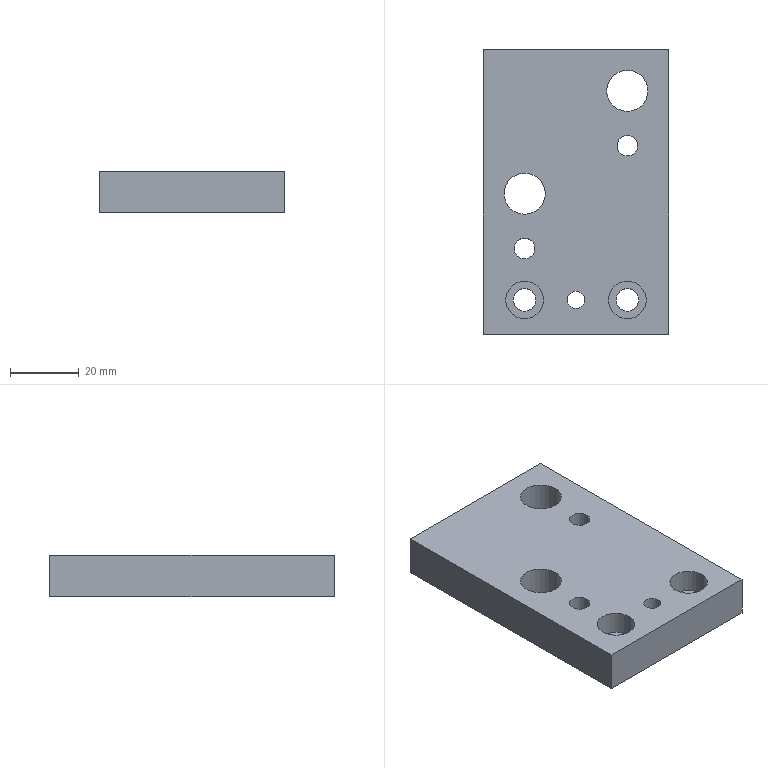Component | NX | DRILL_PLATE | 1 solid | 17 faces | volume 48507 mm3 | cylinder 9 | plane 8 | commonest cylinder face diameters 12 x2 6 x2 6.6 x2 11 x2 5 x1